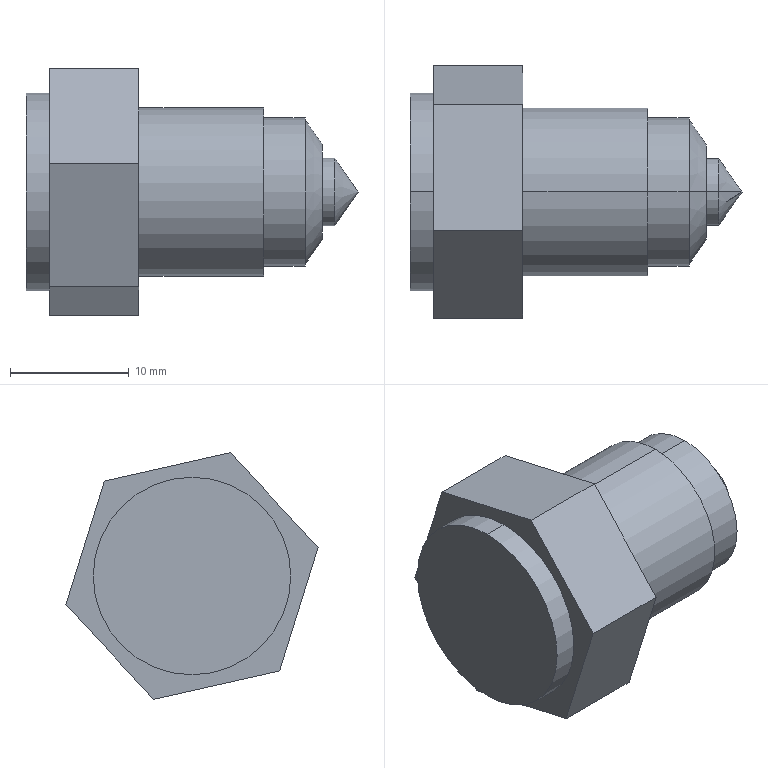Component | SolidWorks | OilCup-2 | 1 solid | 24 faces | box 27.95 x 21.23 x 20.78 mm | volume 4992 mm3 | plane 12 | cylinder 8 | cone 4 | commonest cylinder face diameters 5.676 x2 12.487 x2 14.194 x2 16.633 x2
STEP:
#1=COLOUR_RGB('',0.7922,0.8196,0.9333);
#2=FILL_AREA_STYLE_COLOUR('',#1);
#3=FILL_AREA_STYLE('',(#2));
#4=SURFACE_STYLE_FILL_AREA(#3);
#5=SURFACE_SIDE_STYLE('',(#4));
#6=SURFACE_STYLE_USAGE(.BOTH.,#5);
#7=PRESENTATION_STYLE_ASSIGNMENT((#6));
#8=CARTESIAN_POINT('',(7.784,3.312,-2.737));
#9=VERTEX_POINT('',#8);
#10=CARTESIAN_POINT('',(7.708,3.312,-2.625));
#11=VERTEX_POINT('',#10);
#12=CARTESIAN_POINT('',(7.708,3.312,-2.625));
#13=DIRECTION('',(-0.5656,0.,0.8247));
#14=VECTOR('',#13,39.37);
#15=LINE('',#12,#14);
#16=EDGE_CURVE('',#9,#11,#15,.T.);
#17=ORIENTED_EDGE('',*,*,#16,.F.);
#18=CARTESIAN_POINT('',(7.708,3.312,-2.849));
#19=VERTEX_POINT('',#18);
#20=CARTESIAN_POINT('',(7.708,3.312,-2.849));
#21=DIRECTION('',(-0.5656,0.,-0.8247));
#22=VECTOR('',#21,39.37);
#23=LINE('',#20,#22);
#24=EDGE_CURVE('',#9,#19,#23,.T.);
#25=ORIENTED_EDGE('',*,*,#24,.T.);
#26=CARTESIAN_POINT('',(7.708,3.312,-2.737));
#27=DIRECTION('',(-1.,0.,0.));
#28=DIRECTION('',(0.,0.,1.));
#29=AXIS2_PLACEMENT_3D('',#26,#27,#28);
#30=CIRCLE('',#29,0.1117);
#31=EDGE_CURVE('',#11,#19,#30,.T.);
#32=ORIENTED_EDGE('',*,*,#31,.F.);
#33=EDGE_LOOP('',(#17,#25,#32));
#34=FACE_OUTER_BOUND('',#33,.T.);
#35=CARTESIAN_POINT('',(7.708,3.312,-2.737));
#36=DIRECTION('',(-1.,0.,0.));
#37=DIRECTION('',(0.,0.,1.));
#38=AXIS2_PLACEMENT_3D('',#35,#36,#37);
#39=CONICAL_SURFACE('',#38,0.1117,0.9696);
#40=ADVANCED_FACE('',(#34),#39,.T.);
#41=ORIENTED_EDGE('',*,*,#31,.T.);
#42=CARTESIAN_POINT('',(7.666,3.312,-2.849));
#43=VERTEX_POINT('',#42);
#44=CARTESIAN_POINT('',(7.471,3.312,-2.849));
#45=DIRECTION('',(-1.,0.,0.));
#46=VECTOR('',#45,39.37);
#47=LINE('',#44,#46);
#48=EDGE_CURVE('',#19,#43,#47,.T.);
#49=ORIENTED_EDGE('',*,*,#48,.T.);
#50=CARTESIAN_POINT('',(7.666,3.312,-2.625));
#51=VERTEX_POINT('',#50);
#52=CARTESIAN_POINT('',(7.666,3.312,-2.737));
#53=DIRECTION('',(-1.,0.,0.));
#54=DIRECTION('',(0.,0.,1.));
#55=AXIS2_PLACEMENT_3D('',#52,#53,#54);
#56=CIRCLE('',#55,0.1117);
#57=EDGE_CURVE('',#51,#43,#56,.T.);
#58=ORIENTED_EDGE('',*,*,#57,.F.);
#59=CARTESIAN_POINT('',(7.471,3.312,-2.625));
#60=DIRECTION('',(-1.,0.,0.));
#61=VECTOR('',#60,39.37);
#62=LINE('',#59,#61);
#63=EDGE_CURVE('',#11,#51,#62,.T.);
#64=ORIENTED_EDGE('',*,*,#63,.F.);
#65=EDGE_LOOP('',(#41,#49,#58,#64));
#66=FACE_OUTER_BOUND('',#65,.T.);
#67=CARTESIAN_POINT('',(7.471,3.312,-2.737));
#68=DIRECTION('',(-1.,0.,0.));
#69=DIRECTION('',(0.,0.,1.));
#70=AXIS2_PLACEMENT_3D('',#67,#68,#69);
#71=CYLINDRICAL_SURFACE('',#70,0.1117);
#72=ADVANCED_FACE('',(#66),#71,.T.);
#73=CARTESIAN_POINT('',(7.666,3.312,-2.579));
#74=VERTEX_POINT('',#73);
#75=CARTESIAN_POINT('',(7.666,3.312,-2.895));
#76=VERTEX_POINT('',#75);
#77=CARTESIAN_POINT('',(7.666,3.312,-2.737));
#78=DIRECTION('',(-1.,0.,0.));
#79=DIRECTION('',(0.,0.,1.));
#80=AXIS2_PLACEMENT_3D('',#77,#78,#79);
#81=CIRCLE('',#80,0.1578);
#82=EDGE_CURVE('',#74,#76,#81,.T.);
#83=ORIENTED_EDGE('',*,*,#82,.T.);
#84=CARTESIAN_POINT('',(7.609,3.312,-2.976));
#85=VERTEX_POINT('',#84);
#86=CARTESIAN_POINT('',(7.609,3.312,-2.976));
#87=DIRECTION('',(-0.5753,0.,-0.8179));
#88=VECTOR('',#87,39.37);
#89=LINE('',#86,#88);
#90=EDGE_CURVE('',#76,#85,#89,.T.);
#91=ORIENTED_EDGE('',*,*,#90,.T.);
#92=CARTESIAN_POINT('',(7.609,3.312,-2.498));
#93=VERTEX_POINT('',#92);
#94=CARTESIAN_POINT('',(7.609,3.312,-2.737));
#95=DIRECTION('',(-1.,0.,0.));
#96=DIRECTION('',(0.,0.,1.));
#97=AXIS2_PLACEMENT_3D('',#94,#95,#96);
#98=CIRCLE('',#97,0.239);
#99=EDGE_CURVE('',#93,#85,#98,.T.);
#100=ORIENTED_EDGE('',*,*,#99,.F.);
#101=CARTESIAN_POINT('',(7.609,3.312,-2.498));
#102=DIRECTION('',(-0.5753,0.,0.8179));
#103=VECTOR('',#102,39.37);
#104=LINE('',#101,#103);
#105=EDGE_CURVE('',#74,#93,#104,.T.);
#106=ORIENTED_EDGE('',*,*,#105,.F.);
#107=EDGE_LOOP('',(#83,#91,#100,#106));
#108=FACE_OUTER_BOUND('',#107,.T.);
#109=CARTESIAN_POINT('',(7.609,3.312,-2.737));
#110=DIRECTION('',(-1.,0.,0.));
#111=DIRECTION('',(0.,0.,1.));
#112=AXIS2_PLACEMENT_3D('',#109,#110,#111);
#113=CONICAL_SURFACE('',#112,0.239,0.9578);
#114=ADVANCED_FACE('',(#108),#113,.T.);
#115=CARTESIAN_POINT('',(7.609,3.312,-2.983));
#116=VERTEX_POINT('',#115);
#117=CARTESIAN_POINT('',(7.609,3.312,-2.491));
#118=VERTEX_POINT('',#117);
#119=CARTESIAN_POINT('',(7.609,3.312,-2.737));
#120=DIRECTION('',(1.,-0.,-0.));
#121=DIRECTION('',(0.,0.,-1.));
#122=AXIS2_PLACEMENT_3D('',#119,#120,#121);
#123=CIRCLE('',#122,0.2458);
#124=EDGE_CURVE('',#116,#118,#123,.T.);
#125=ORIENTED_EDGE('',*,*,#124,.F.);
#126=CARTESIAN_POINT('',(7.471,3.312,-2.983));
#127=VERTEX_POINT('',#126);
#128=CARTESIAN_POINT('',(7.609,3.312,-2.983));
#129=DIRECTION('',(-1.,0.,0.));
#130=VECTOR('',#129,39.37);
#131=LINE('',#128,#130);
#132=EDGE_CURVE('',#116,#127,#131,.T.);
#133=ORIENTED_EDGE('',*,*,#132,.T.);
#134=CARTESIAN_POINT('',(7.471,3.312,-2.491));
#135=VERTEX_POINT('',#134);
#136=CARTESIAN_POINT('',(7.471,3.312,-2.737));
#137=DIRECTION('',(1.,-0.,-0.));
#138=DIRECTION('',(0.,0.,-1.));
#139=AXIS2_PLACEMENT_3D('',#136,#137,#138);
#140=CIRCLE('',#139,0.2458);
#141=EDGE_CURVE('',#127,#135,#140,.T.);
#142=ORIENTED_EDGE('',*,*,#141,.T.);
#143=CARTESIAN_POINT('',(7.609,3.312,-2.491));
#144=DIRECTION('',(-1.,0.,0.));
#145=VECTOR('',#144,39.37);
#146=LINE('',#143,#145);
#147=EDGE_CURVE('',#118,#135,#146,.T.);
#148=ORIENTED_EDGE('',*,*,#147,.F.);
#149=EDGE_LOOP('',(#125,#133,#142,#148));
#150=FACE_OUTER_BOUND('',#149,.T.);
#151=CARTESIAN_POINT('',(7.609,3.312,-2.737));
#152=DIRECTION('',(-1.,0.,0.));
#153=DIRECTION('',(0.,0.,1.));
#154=AXIS2_PLACEMENT_3D('',#151,#152,#153);
#155=CYLINDRICAL_SURFACE('',#154,0.2458);
#156=ADVANCED_FACE('',(#150),#155,.T.);
#157=CARTESIAN_POINT('',(7.471,3.312,-3.016));
#158=VERTEX_POINT('',#157);
#159=CARTESIAN_POINT('',(7.471,3.312,-2.457));
#160=VERTEX_POINT('',#159);
#161=CARTESIAN_POINT('',(7.471,3.312,-2.737));
#162=DIRECTION('',(1.,-0.,-0.));
#163=DIRECTION('',(0.,0.,-1.));
#164=AXIS2_PLACEMENT_3D('',#161,#162,#163);
#165=CIRCLE('',#164,0.2794);
#166=EDGE_CURVE('',#158,#160,#165,.T.);
#167=ORIENTED_EDGE('',*,*,#166,.F.);
#168=CARTESIAN_POINT('',(7.058,3.312,-3.016));
#169=VERTEX_POINT('',#168);
#170=CARTESIAN_POINT('',(7.471,3.312,-3.016));
#171=DIRECTION('',(-1.,0.,0.));
#172=VECTOR('',#171,39.37);
#173=LINE('',#170,#172);
#174=EDGE_CURVE('',#158,#169,#173,.T.);
#175=ORIENTED_EDGE('',*,*,#174,.T.);
#176=CARTESIAN_POINT('',(7.058,3.312,-2.457));
#177=VERTEX_POINT('',#176);
#178=CARTESIAN_POINT('',(7.058,3.312,-2.737));
#179=DIRECTION('',(1.,-0.,-0.));
#180=DIRECTION('',(0.,0.,-1.));
#181=AXIS2_PLACEMENT_3D('',#178,#179,#180);
#182=CIRCLE('',#181,0.2794);
#183=EDGE_CURVE('',#169,#177,#182,.T.);
#184=ORIENTED_EDGE('',*,*,#183,.T.);
#185=CARTESIAN_POINT('',(7.471,3.312,-2.457));
#186=DIRECTION('',(-1.,0.,0.));
#187=VECTOR('',#186,39.37);
#188=LINE('',#185,#187);
#189=EDGE_CURVE('',#160,#177,#188,.T.);
#190=ORIENTED_EDGE('',*,*,#189,.F.);
#191=EDGE_LOOP('',(#167,#175,#184,#190));
#192=FACE_OUTER_BOUND('',#191,.T.);
#193=CARTESIAN_POINT('',(7.471,3.312,-2.737));
#194=DIRECTION('',(-1.,0.,0.));
#195=DIRECTION('',(0.,0.,1.));
#196=AXIS2_PLACEMENT_3D('',#193,#194,#195);
#197=CYLINDRICAL_SURFACE('',#196,0.2794);
#198=ADVANCED_FACE('',(#192),#197,.T.);
#199=CARTESIAN_POINT('',(6.763,3.312,-3.064));
#200=VERTEX_POINT('',#199);
#201=CARTESIAN_POINT('',(6.763,3.312,-2.409));
#202=VERTEX_POINT('',#201);
#203=CARTESIAN_POINT('',(6.763,3.312,-2.737));
#204=DIRECTION('',(1.,-0.,-0.));
#205=DIRECTION('',(0.,0.,-1.));
#206=AXIS2_PLACEMENT_3D('',#203,#204,#205);
#207=CIRCLE('',#206,0.3274);
#208=EDGE_CURVE('',#200,#202,#207,.T.);
#209=ORIENTED_EDGE('',*,*,#208,.F.);
#210=CARTESIAN_POINT('',(6.684,3.312,-3.064));
#211=VERTEX_POINT('',#210);
#212=CARTESIAN_POINT('',(7.058,3.312,-3.064));
#213=DIRECTION('',(-1.,0.,0.));
#214=VECTOR('',#213,39.37);
#215=LINE('',#212,#214);
#216=EDGE_CURVE('',#200,#211,#215,.T.);
#217=ORIENTED_EDGE('',*,*,#216,.T.);
#218=CARTESIAN_POINT('',(6.684,3.312,-2.409));
#219=VERTEX_POINT('',#218);
#220=CARTESIAN_POINT('',(6.684,3.312,-2.737));
#221=DIRECTION('',(1.,-0.,-0.));
#222=DIRECTION('',(0.,0.,-1.));
#223=AXIS2_PLACEMENT_3D('',#220,#221,#222);
#224=CIRCLE('',#223,0.3274);
#225=EDGE_CURVE('',#211,#219,#224,.T.);
#226=ORIENTED_EDGE('',*,*,#225,.T.);
#227=CARTESIAN_POINT('',(7.058,3.312,-2.409));
#228=DIRECTION('',(-1.,0.,0.));
#229=VECTOR('',#228,39.37);
#230=LINE('',#227,#229);
#231=EDGE_CURVE('',#202,#219,#230,.T.);
#232=ORIENTED_EDGE('',*,*,#231,.F.);
#233=EDGE_LOOP('',(#209,#217,#226,#232));
#234=FACE_OUTER_BOUND('',#233,.T.);
#235=CARTESIAN_POINT('',(7.058,3.312,-2.737));
#236=DIRECTION('',(-1.,0.,0.));
#237=DIRECTION('',(0.,0.,1.));
#238=AXIS2_PLACEMENT_3D('',#235,#236,#237);
#239=CYLINDRICAL_SURFACE('',#238,0.3274);
#240=ADVANCED_FACE('',(#234),#239,.T.);
#241=ORIENTED_EDGE('',*,*,#216,.F.);
#242=CARTESIAN_POINT('',(6.763,3.312,-2.737));
#243=DIRECTION('',(1.,-0.,-0.));
#244=DIRECTION('',(0.,0.,-1.));
#245=AXIS2_PLACEMENT_3D('',#242,#243,#244);
#246=CIRCLE('',#245,0.3274);
#247=EDGE_CURVE('',#202,#200,#246,.T.);
#248=ORIENTED_EDGE('',*,*,#247,.F.);
#249=ORIENTED_EDGE('',*,*,#231,.T.);
#250=CARTESIAN_POINT('',(6.684,3.312,-2.737));
#251=DIRECTION('',(1.,-0.,-0.));
#252=DIRECTION('',(0.,0.,-1.));
#253=AXIS2_PLACEMENT_3D('',#250,#251,#252);
#254=CIRCLE('',#253,0.3274);
#255=EDGE_CURVE('',#219,#211,#254,.T.);
#256=ORIENTED_EDGE('',*,*,#255,.T.);
#257=EDGE_LOOP('',(#241,#248,#249,#256));
#258=FACE_OUTER_BOUND('',#257,.T.);
#259=CARTESIAN_POINT('',(7.058,3.312,-2.737));
#260=DIRECTION('',(-1.,0.,0.));
#261=DIRECTION('',(0.,0.,1.));
#262=AXIS2_PLACEMENT_3D('',#259,#260,#261);
#263=CYLINDRICAL_SURFACE('',#262,0.3274);
#264=ADVANCED_FACE('',(#258),#263,.T.);
#265=ORIENTED_EDGE('',*,*,#255,.F.);
#266=ORIENTED_EDGE('',*,*,#225,.F.);
#267=EDGE_LOOP('',(#265,#266));
#268=FACE_OUTER_BOUND('',#267,.T.);
#269=CARTESIAN_POINT('',(6.684,3.312,-2.737));
#270=DIRECTION('',(1.,-0.,-0.));
#271=DIRECTION('',(-0.,0.,-1.));
#272=AXIS2_PLACEMENT_3D('',#269,#270,#271);
#273=PLANE('',#272);
#274=ADVANCED_FACE('',(#268),#273,.F.);
#275=CARTESIAN_POINT('',(7.058,3.439,-3.146));
#276=VERTEX_POINT('',#275);
#277=CARTESIAN_POINT('',(7.058,3.729,-2.831));
#278=VERTEX_POINT('',#277);
#279=CARTESIAN_POINT('',(7.058,3.439,-3.146));
#280=DIRECTION('',(0.,0.6784,0.7347));
#281=VECTOR('',#280,39.37);
#282=LINE('',#279,#281);
#283=EDGE_CURVE('',#276,#278,#282,.T.);
#284=ORIENTED_EDGE('',*,*,#283,.F.);
#285=CARTESIAN_POINT('',(6.763,3.439,-3.146));
#286=VERTEX_POINT('',#285);
#287=CARTESIAN_POINT('',(6.763,3.439,-3.146));
#288=DIRECTION('',(1.,-0.,-0.));
#289=VECTOR('',#288,39.37);
#290=LINE('',#287,#289);
#291=EDGE_CURVE('',#286,#276,#290,.T.);
#292=ORIENTED_EDGE('',*,*,#291,.F.);
#293=CARTESIAN_POINT('',(6.763,3.729,-2.831));
#294=VERTEX_POINT('',#293);
#295=CARTESIAN_POINT('',(6.763,3.439,-3.146));
#296=DIRECTION('',(0.,0.6784,0.7347));
#297=VECTOR('',#296,39.37);
#298=LINE('',#295,#297);
#299=EDGE_CURVE('',#286,#294,#298,.T.);
#300=ORIENTED_EDGE('',*,*,#299,.T.);
#301=CARTESIAN_POINT('',(6.763,3.729,-2.831));
#302=DIRECTION('',(1.,-0.,-0.));
#303=VECTOR('',#302,39.37);
#304=LINE('',#301,#303);
#305=EDGE_CURVE('',#294,#278,#304,.T.);
#306=ORIENTED_EDGE('',*,*,#305,.T.);
#307=EDGE_LOOP('',(#284,#292,#300,#306));
#308=FACE_OUTER_BOUND('',#307,.T.);
#309=CARTESIAN_POINT('',(6.763,3.439,-3.146));
#310=DIRECTION('',(0.,0.7347,-0.6784));
#311=DIRECTION('',(0.,0.6784,0.7347));
#312=AXIS2_PLACEMENT_3D('',#309,#310,#311);
#313=PLANE('',#312);
#314=ADVANCED_FACE('',(#308),#313,.T.);
#315=CARTESIAN_POINT('',(7.058,3.021,-3.052));
#316=VERTEX_POINT('',#315);
#317=CARTESIAN_POINT('',(7.058,3.021,-3.052));
#318=DIRECTION('',(0.,0.9755,-0.2202));
#319=VECTOR('',#318,39.37);
#320=LINE('',#317,#319);
#321=EDGE_CURVE('',#316,#276,#320,.T.);
#322=ORIENTED_EDGE('',*,*,#321,.F.);
#323=CARTESIAN_POINT('',(6.763,3.021,-3.052));
#324=VERTEX_POINT('',#323);
#325=CARTESIAN_POINT('',(6.763,3.021,-3.052));
#326=DIRECTION('',(1.,-0.,-0.));
#327=VECTOR('',#326,39.37);
#328=LINE('',#325,#327);
#329=EDGE_CURVE('',#324,#316,#328,.T.);
#330=ORIENTED_EDGE('',*,*,#329,.F.);
#331=CARTESIAN_POINT('',(6.763,3.021,-3.052));
#332=DIRECTION('',(0.,0.9755,-0.2202));
#333=VECTOR('',#332,39.37);
#334=LINE('',#331,#333);
#335=EDGE_CURVE('',#324,#286,#334,.T.);
#336=ORIENTED_EDGE('',*,*,#335,.T.);
#337=ORIENTED_EDGE('',*,*,#291,.T.);
#338=EDGE_LOOP('',(#322,#330,#336,#337));
#339=FACE_OUTER_BOUND('',#338,.T.);
#340=CARTESIAN_POINT('',(6.763,3.021,-3.052));
#341=DIRECTION('',(-0.,-0.2202,-0.9755));
#342=DIRECTION('',(0.,0.9755,-0.2202));
#343=AXIS2_PLACEMENT_3D('',#340,#341,#342);
#344=PLANE('',#343);
#345=ADVANCED_FACE('',(#339),#344,.T.);
#346=CARTESIAN_POINT('',(7.058,2.894,-2.643));
#347=VERTEX_POINT('',#346);
#348=CARTESIAN_POINT('',(7.058,2.894,-2.643));
#349=DIRECTION('',(-0.,0.297,-0.9549));
#350=VECTOR('',#349,39.37);
#351=LINE('',#348,#350);
#352=EDGE_CURVE('',#347,#316,#351,.T.);
#353=ORIENTED_EDGE('',*,*,#352,.F.);
#354=CARTESIAN_POINT('',(6.763,2.894,-2.643));
#355=VERTEX_POINT('',#354);
#356=CARTESIAN_POINT('',(6.763,2.894,-2.643));
#357=DIRECTION('',(1.,-0.,-0.));
#358=VECTOR('',#357,39.37);
#359=LINE('',#356,#358);
#360=EDGE_CURVE('',#355,#347,#359,.T.);
#361=ORIENTED_EDGE('',*,*,#360,.F.);
#362=CARTESIAN_POINT('',(6.763,2.894,-2.643));
#363=DIRECTION('',(-0.,0.297,-0.9549));
#364=VECTOR('',#363,39.37);
#365=LINE('',#362,#364);
#366=EDGE_CURVE('',#355,#324,#365,.T.);
#367=ORIENTED_EDGE('',*,*,#366,.T.);
#368=ORIENTED_EDGE('',*,*,#329,.T.);
#369=EDGE_LOOP('',(#353,#361,#367,#368));
#370=FACE_OUTER_BOUND('',#369,.T.);
#371=CARTESIAN_POINT('',(6.763,2.894,-2.643));
#372=DIRECTION('',(-0.,-0.9549,-0.297));
#373=DIRECTION('',(-0.,0.297,-0.9549));
#374=AXIS2_PLACEMENT_3D('',#371,#372,#373);
#375=PLANE('',#374);
#376=ADVANCED_FACE('',(#370),#375,.T.);
#377=CARTESIAN_POINT('',(7.058,3.184,-2.328));
#378=VERTEX_POINT('',#377);
#379=CARTESIAN_POINT('',(7.058,3.184,-2.328));
#380=DIRECTION('',(-0.,-0.6784,-0.7347));
#381=VECTOR('',#380,39.37);
#382=LINE('',#379,#381);
#383=EDGE_CURVE('',#378,#347,#382,.T.);
#384=ORIENTED_EDGE('',*,*,#383,.F.);
#385=CARTESIAN_POINT('',(6.763,3.184,-2.328));
#386=VERTEX_POINT('',#385);
#387=CARTESIAN_POINT('',(6.763,3.184,-2.328));
#388=DIRECTION('',(1.,-0.,-0.));
#389=VECTOR('',#388,39.37);
#390=LINE('',#387,#389);
#391=EDGE_CURVE('',#386,#378,#390,.T.);
#392=ORIENTED_EDGE('',*,*,#391,.F.);
#393=CARTESIAN_POINT('',(6.763,3.184,-2.328));
#394=DIRECTION('',(-0.,-0.6784,-0.7347));
#395=VECTOR('',#394,39.37);
#396=LINE('',#393,#395);
#397=EDGE_CURVE('',#386,#355,#396,.T.);
#398=ORIENTED_EDGE('',*,*,#397,.T.);
#399=ORIENTED_EDGE('',*,*,#360,.T.);
#400=EDGE_LOOP('',(#384,#392,#398,#399));
#401=FACE_OUTER_BOUND('',#400,.T.);
#402=CARTESIAN_POINT('',(6.763,3.184,-2.328));
#403=DIRECTION('',(-0.,-0.7347,0.6784));
#404=DIRECTION('',(-0.,-0.6784,-0.7347));
#405=AXIS2_PLACEMENT_3D('',#402,#403,#404);
#406=PLANE('',#405);
#407=ADVANCED_FACE('',(#401),#406,.T.);
#408=CARTESIAN_POINT('',(7.058,3.602,-2.422));
#409=VERTEX_POINT('',#408);
#410=CARTESIAN_POINT('',(7.058,3.602,-2.422));
#411=DIRECTION('',(-0.,-0.9755,0.2202));
#412=VECTOR('',#411,39.37);
#413=LINE('',#410,#412);
#414=EDGE_CURVE('',#409,#378,#413,.T.);
#415=ORIENTED_EDGE('',*,*,#414,.F.);
#416=CARTESIAN_POINT('',(6.763,3.602,-2.422));
#417=VERTEX_POINT('',#416);
#418=CARTESIAN_POINT('',(6.763,3.602,-2.422));
#419=DIRECTION('',(1.,-0.,-0.));
#420=VECTOR('',#419,39.37);
#421=LINE('',#418,#420);
#422=EDGE_CURVE('',#417,#409,#421,.T.);
#423=ORIENTED_EDGE('',*,*,#422,.F.);
#424=CARTESIAN_POINT('',(6.763,3.602,-2.422));
#425=DIRECTION('',(-0.,-0.9755,0.2202));
#426=VECTOR('',#425,39.37);
#427=LINE('',#424,#426);
#428=EDGE_CURVE('',#417,#386,#427,.T.);
#429=ORIENTED_EDGE('',*,*,#428,.T.);
#430=ORIENTED_EDGE('',*,*,#391,.T.);
#431=EDGE_LOOP('',(#415,#423,#429,#430));
#432=FACE_OUTER_BOUND('',#431,.T.);
#433=CARTESIAN_POINT('',(6.763,3.602,-2.422));
#434=DIRECTION('',(0.,0.2202,0.9755));
#435=DIRECTION('',(-0.,-0.9755,0.2202));
#436=AXIS2_PLACEMENT_3D('',#433,#434,#435);
#437=PLANE('',#436);
#438=ADVANCED_FACE('',(#432),#437,.T.);
#439=CARTESIAN_POINT('',(7.058,3.729,-2.831));
#440=DIRECTION('',(0.,-0.297,0.9549));
#441=VECTOR('',#440,39.37);
#442=LINE('',#439,#441);
#443=EDGE_CURVE('',#278,#409,#442,.T.);
#444=ORIENTED_EDGE('',*,*,#443,.F.);
#445=ORIENTED_EDGE('',*,*,#305,.F.);
#446=CARTESIAN_POINT('',(6.763,3.729,-2.831));
#447=DIRECTION('',(0.,-0.297,0.9549));
#448=VECTOR('',#447,39.37);
#449=LINE('',#446,#448);
#450=EDGE_CURVE('',#294,#417,#449,.T.);
#451=ORIENTED_EDGE('',*,*,#450,.T.);
#452=ORIENTED_EDGE('',*,*,#422,.T.);
#453=EDGE_LOOP('',(#444,#445,#451,#452));
#454=FACE_OUTER_BOUND('',#453,.T.);
#455=CARTESIAN_POINT('',(6.763,3.729,-2.831));
#456=DIRECTION('',(0.,0.9549,0.297));
#457=DIRECTION('',(0.,-0.297,0.9549));
#458=AXIS2_PLACEMENT_3D('',#455,#456,#457);
#459=PLANE('',#458);
#460=ADVANCED_FACE('',(#454),#459,.T.);
#461=ORIENTED_EDGE('',*,*,#247,.T.);
#462=ORIENTED_EDGE('',*,*,#208,.T.);
#463=EDGE_LOOP('',(#461,#462));
#464=FACE_BOUND('',#463,.T.);
#465=ORIENTED_EDGE('',*,*,#299,.F.);
#466=ORIENTED_EDGE('',*,*,#335,.F.);
#467=ORIENTED_EDGE('',*,*,#366,.F.);
#468=ORIENTED_EDGE('',*,*,#397,.F.);
#469=ORIENTED_EDGE('',*,*,#428,.F.);
#470=ORIENTED_EDGE('',*,*,#450,.F.);
#471=EDGE_LOOP('',(#465,#466,#467,#468,#469,#470));
#472=FACE_OUTER_BOUND('',#471,.T.);
#473=CARTESIAN_POINT('',(6.763,3.333,-0.06872));
#474=DIRECTION('',(1.,-0.,-0.));
#475=DIRECTION('',(-0.,0.,-1.));
#476=AXIS2_PLACEMENT_3D('',#473,#474,#475);
#477=PLANE('',#476);
#478=ADVANCED_FACE('',(#464,#472),#477,.F.);
#479=CARTESIAN_POINT('',(7.058,3.312,-2.737));
#480=DIRECTION('',(1.,-0.,-0.));
#481=DIRECTION('',(0.,0.,-1.));
#482=AXIS2_PLACEMENT_3D('',#479,#480,#481);
#483=CIRCLE('',#482,0.2794);
#484=EDGE_CURVE('',#177,#169,#483,.T.);
#485=ORIENTED_EDGE('',*,*,#484,.F.);
#486=ORIENTED_EDGE('',*,*,#183,.F.);
#487=EDGE_LOOP('',(#485,#486));
#488=FACE_BOUND('',#487,.T.);
#489=ORIENTED_EDGE('',*,*,#283,.T.);
#490=ORIENTED_EDGE('',*,*,#443,.T.);
#491=ORIENTED_EDGE('',*,*,#414,.T.);
#492=ORIENTED_EDGE('',*,*,#383,.T.);
#493=ORIENTED_EDGE('',*,*,#352,.T.);
#494=ORIENTED_EDGE('',*,*,#321,.T.);
#495=EDGE_LOOP('',(#489,#490,#491,#492,#493,#494));
#496=FACE_OUTER_BOUND('',#495,.T.);
#497=CARTESIAN_POINT('',(7.058,3.312,-2.737));
#498=DIRECTION('',(1.,-0.,-0.));
#499=DIRECTION('',(-0.,0.,-1.));
#500=AXIS2_PLACEMENT_3D('',#497,#498,#499);
#501=PLANE('',#500);
#502=ADVANCED_FACE('',(#488,#496),#501,.T.);
#503=ORIENTED_EDGE('',*,*,#174,.F.);
#504=CARTESIAN_POINT('',(7.471,3.312,-2.737));
#505=DIRECTION('',(1.,-0.,-0.));
#506=DIRECTION('',(0.,0.,-1.));
#507=AXIS2_PLACEMENT_3D('',#504,#505,#506);
#508=CIRCLE('',#507,0.2794);
#509=EDGE_CURVE('',#160,#158,#508,.T.);
#510=ORIENTED_EDGE('',*,*,#509,.F.);
#511=ORIENTED_EDGE('',*,*,#189,.T.);
#512=ORIENTED_EDGE('',*,*,#484,.T.);
#513=EDGE_LOOP('',(#503,#510,#511,#512));
#514=FACE_OUTER_BOUND('',#513,.T.);
#515=CARTESIAN_POINT('',(7.471,3.312,-2.737));
#516=DIRECTION('',(-1.,0.,0.));
#517=DIRECTION('',(0.,0.,1.));
#518=AXIS2_PLACEMENT_3D('',#515,#516,#517);
#519=CYLINDRICAL_SURFACE('',#518,0.2794);
#520=ADVANCED_FACE('',(#514),#519,.T.);
#521=CARTESIAN_POINT('',(7.471,3.312,-2.737));
#522=DIRECTION('',(1.,-0.,-0.));
#523=DIRECTION('',(0.,0.,-1.));
#524=AXIS2_PLACEMENT_3D('',#521,#522,#523);
#525=CIRCLE('',#524,0.2458);
#526=EDGE_CURVE('',#135,#127,#525,.T.);
#527=ORIENTED_EDGE('',*,*,#526,.F.);
#528=ORIENTED_EDGE('',*,*,#141,.F.);
#529=EDGE_LOOP('',(#527,#528));
#530=FACE_BOUND('',#529,.T.);
#531=ORIENTED_EDGE('',*,*,#509,.T.);
#532=ORIENTED_EDGE('',*,*,#166,.T.);
#533=EDGE_LOOP('',(#531,#532));
#534=FACE_OUTER_BOUND('',#533,.T.);
#535=CARTESIAN_POINT('',(7.471,3.312,-2.737));
#536=DIRECTION('',(1.,-0.,-0.));
#537=DIRECTION('',(-0.,0.,-1.));
#538=AXIS2_PLACEMENT_3D('',#535,#536,#537);
#539=PLANE('',#538);
#540=ADVANCED_FACE('',(#530,#534),#539,.T.);
#541=ORIENTED_EDGE('',*,*,#132,.F.);
#542=CARTESIAN_POINT('',(7.609,3.312,-2.737));
#543=DIRECTION('',(1.,-0.,-0.));
#544=DIRECTION('',(0.,0.,-1.));
#545=AXIS2_PLACEMENT_3D('',#542,#543,#544);
#546=CIRCLE('',#545,0.2458);
#547=EDGE_CURVE('',#118,#116,#546,.T.);
#548=ORIENTED_EDGE('',*,*,#547,.F.);
#549=ORIENTED_EDGE('',*,*,#147,.T.);
#550=ORIENTED_EDGE('',*,*,#526,.T.);
#551=EDGE_LOOP('',(#541,#548,#549,#550));
#552=FACE_OUTER_BOUND('',#551,.T.);
#553=CARTESIAN_POINT('',(7.609,3.312,-2.737));
#554=DIRECTION('',(-1.,0.,0.));
#555=DIRECTION('',(0.,0.,1.));
#556=AXIS2_PLACEMENT_3D('',#553,#554,#555);
#557=CYLINDRICAL_SURFACE('',#556,0.2458);
#558=ADVANCED_FACE('',(#552),#557,.T.);
#559=ORIENTED_EDGE('',*,*,#99,.T.);
#560=CARTESIAN_POINT('',(7.609,3.312,-2.737));
#561=DIRECTION('',(-1.,0.,0.));
#562=DIRECTION('',(0.,0.,1.));
#563=AXIS2_PLACEMENT_3D('',#560,#561,#562);
#564=CIRCLE('',#563,0.239);
#565=EDGE_CURVE('',#85,#93,#564,.T.);
#566=ORIENTED_EDGE('',*,*,#565,.T.);
#567=EDGE_LOOP('',(#559,#566));
#568=FACE_BOUND('',#567,.T.);
#569=ORIENTED_EDGE('',*,*,#547,.T.);
#570=ORIENTED_EDGE('',*,*,#124,.T.);
#571=EDGE_LOOP('',(#569,#570));
#572=FACE_OUTER_BOUND('',#571,.T.);
#573=CARTESIAN_POINT('',(7.609,3.312,-2.737));
#574=DIRECTION('',(1.,-0.,-0.));
#575=DIRECTION('',(-0.,0.,-1.));
#576=AXIS2_PLACEMENT_3D('',#573,#574,#575);
#577=PLANE('',#576);
#578=ADVANCED_FACE('',(#568,#572),#577,.T.);
#579=ORIENTED_EDGE('',*,*,#90,.F.);
#580=CARTESIAN_POINT('',(7.666,3.312,-2.737));
#581=DIRECTION('',(-1.,0.,0.));
#582=DIRECTION('',(0.,0.,1.));
#583=AXIS2_PLACEMENT_3D('',#580,#581,#582);
#584=CIRCLE('',#583,0.1578);
#585=EDGE_CURVE('',#76,#74,#584,.T.);
#586=ORIENTED_EDGE('',*,*,#585,.T.);
#587=ORIENTED_EDGE('',*,*,#105,.T.);
#588=ORIENTED_EDGE('',*,*,#565,.F.);
#589=EDGE_LOOP('',(#579,#586,#587,#588));
#590=FACE_OUTER_BOUND('',#589,.T.);
#591=CARTESIAN_POINT('',(7.609,3.312,-2.737));
#592=DIRECTION('',(-1.,0.,0.));
#593=DIRECTION('',(0.,0.,1.));
#594=AXIS2_PLACEMENT_3D('',#591,#592,#593);
#595=CONICAL_SURFACE('',#594,0.239,0.9578);
#596=ADVANCED_FACE('',(#590),#595,.T.);
#597=ORIENTED_EDGE('',*,*,#57,.T.);
#598=CARTESIAN_POINT('',(7.666,3.312,-2.737));
#599=DIRECTION('',(-1.,0.,0.));
#600=DIRECTION('',(0.,0.,1.));
#601=AXIS2_PLACEMENT_3D('',#598,#599,#600);
#602=CIRCLE('',#601,0.1117);
#603=EDGE_CURVE('',#43,#51,#602,.T.);
#604=ORIENTED_EDGE('',*,*,#603,.T.);
#605=EDGE_LOOP('',(#597,#604));
#606=FACE_BOUND('',#605,.T.);
#607=ORIENTED_EDGE('',*,*,#82,.F.);
#608=ORIENTED_EDGE('',*,*,#585,.F.);
#609=EDGE_LOOP('',(#607,#608));
#610=FACE_OUTER_BOUND('',#609,.T.);
#611=CARTESIAN_POINT('',(7.666,2.557,-0.3102));
#612=DIRECTION('',(1.,-0.,-0.));
#613=DIRECTION('',(-0.,0.,-1.));
#614=AXIS2_PLACEMENT_3D('',#611,#612,#613);
#615=PLANE('',#614);
#616=ADVANCED_FACE('',(#606,#610),#615,.T.);
#617=ORIENTED_EDGE('',*,*,#48,.F.);
#618=CARTESIAN_POINT('',(7.708,3.312,-2.737));
#619=DIRECTION('',(-1.,0.,0.));
#620=DIRECTION('',(0.,0.,1.));
#621=AXIS2_PLACEMENT_3D('',#618,#619,#620);
#622=CIRCLE('',#621,0.1117);
#623=EDGE_CURVE('',#19,#11,#622,.T.);
#624=ORIENTED_EDGE('',*,*,#623,.T.);
#625=ORIENTED_EDGE('',*,*,#63,.T.);
#626=ORIENTED_EDGE('',*,*,#603,.F.);
#627=EDGE_LOOP('',(#617,#624,#625,#626));
#628=FACE_OUTER_BOUND('',#627,.T.);
#629=CARTESIAN_POINT('',(7.471,3.312,-2.737));
#630=DIRECTION('',(-1.,0.,0.));
#631=DIRECTION('',(0.,0.,1.));
#632=AXIS2_PLACEMENT_3D('',#629,#630,#631);
#633=CYLINDRICAL_SURFACE('',#632,0.1117);
#634=ADVANCED_FACE('',(#628),#633,.T.);
#635=ORIENTED_EDGE('',*,*,#24,.F.);
#636=ORIENTED_EDGE('',*,*,#16,.T.);
#637=ORIENTED_EDGE('',*,*,#623,.F.);
#638=EDGE_LOOP('',(#635,#636,#637));
#639=FACE_OUTER_BOUND('',#638,.T.);
#640=CARTESIAN_POINT('',(7.708,3.312,-2.737));
#641=DIRECTION('',(-1.,0.,0.));
#642=DIRECTION('',(0.,0.,1.));
#643=AXIS2_PLACEMENT_3D('',#640,#641,#642);
#644=CONICAL_SURFACE('',#643,0.1117,0.9696);
#645=ADVANCED_FACE('',(#639),#644,.T.);
#646=CLOSED_SHELL('',(#40,#72,#114,#156,#198,#240,#264,#274,#314,#345,#376,#407,#438,#460,#478,#502,#520,#540,#558,#578,#596,#616,#634,#645));
#647=MANIFOLD_SOLID_BREP('',#646);
#648=STYLED_ITEM('',(#7),#647);
#649=PRESENTATION_LAYER_ASSIGNMENT('','',(#648));
#650=(LENGTH_UNIT()NAMED_UNIT(*)SI_UNIT($,.METRE.));
#651=LENGTH_MEASURE_WITH_UNIT(LENGTH_MEASURE(0.0254),#650);
#652=DIMENSIONAL_EXPONENTS(1.,0.,0.,0.,0.,0.,0.);
#653=(CONVERSION_BASED_UNIT('',#651)LENGTH_UNIT()NAMED_UNIT(#652));
#654=UNCERTAINTY_MEASURE_WITH_UNIT(LENGTH_MEASURE(0.00001),#653,'','');
#655=(NAMED_UNIT(*)PLANE_ANGLE_UNIT()SI_UNIT($,.RADIAN.));
#656=(NAMED_UNIT(*)SI_UNIT($,.STERADIAN.)SOLID_ANGLE_UNIT());
#657=(GEOMETRIC_REPRESENTATION_CONTEXT(3)GLOBAL_UNCERTAINTY_ASSIGNED_CONTEXT((#654))GLOBAL_UNIT_ASSIGNED_CONTEXT((#653,#655,#656))REPRESENTATION_CONTEXT('',''));
#658=MECHANICAL_DESIGN_GEOMETRIC_PRESENTATION_REPRESENTATION('',(#648),#657);
#659=CARTESIAN_POINT('',(0.,0.,0.));
#660=DIRECTION('',(0.,0.,1.));
#661=DIRECTION('',(1.,0.,0.));
#662=AXIS2_PLACEMENT_3D('',#659,#660,#661);
#663=(LENGTH_UNIT()NAMED_UNIT(*)SI_UNIT($,.METRE.));
#664=LENGTH_MEASURE_WITH_UNIT(LENGTH_MEASURE(0.0254),#663);
#665=DIMENSIONAL_EXPONENTS(1.,0.,0.,0.,0.,0.,0.);
#666=(CONVERSION_BASED_UNIT('',#664)LENGTH_UNIT()NAMED_UNIT(#665));
#667=UNCERTAINTY_MEASURE_WITH_UNIT(LENGTH_MEASURE(0.00001),#666,'','');
#668=(NAMED_UNIT(*)PLANE_ANGLE_UNIT()SI_UNIT($,.RADIAN.));
#669=(NAMED_UNIT(*)SI_UNIT($,.STERADIAN.)SOLID_ANGLE_UNIT());
#670=(GEOMETRIC_REPRESENTATION_CONTEXT(3)GLOBAL_UNCERTAINTY_ASSIGNED_CONTEXT((#667))GLOBAL_UNIT_ASSIGNED_CONTEXT((#666,#668,#669))REPRESENTATION_CONTEXT('',''));
#671=ADVANCED_BREP_SHAPE_REPRESENTATION('',(#647,#662),#670);